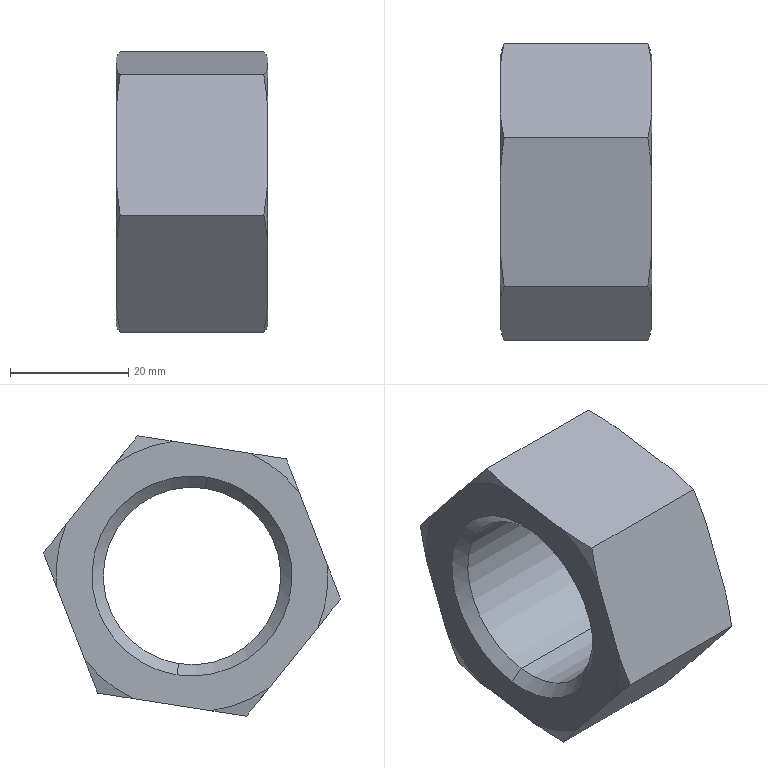Component | SolidWorks | 13Type1HexNut_FinePitch_GradeAAndB[GBT6171-2000][M30_2]-2 | 1 solid | 26 faces | box 25.6 x 50.25 x 47.42 mm | volume 24510 mm3 | cone 16 | plane 8 | cylinder 2 | commonest cylinder face diameters 30 x2 | material Steel
STEP:
#1=CARTESIAN_POINT('',(9.354,-3.462,19.574));
#2=VERTEX_POINT('',#1);
#3=CARTESIAN_POINT('',(9.354,-3.639,20.741));
#4=VERTEX_POINT('',#3);
#5=CARTESIAN_POINT('',(9.354,-3.551,20.157));
#6=DIRECTION('',(-1.,0.,0.));
#7=DIRECTION('',(0.,-0.1496,0.9887));
#8=AXIS2_PLACEMENT_3D('',#5,#6,#7);
#9=CIRCLE('',#8,0.5906);
#10=EDGE_CURVE('',#2,#4,#9,.T.);
#11=ORIENTED_EDGE('',*,*,#10,.F.);
#12=CARTESIAN_POINT('',(9.279,-3.451,19.499));
#13=VERTEX_POINT('',#12);
#14=CARTESIAN_POINT('',(9.354,-3.462,19.574));
#15=DIRECTION('',(-0.7071,0.1058,-0.6991));
#16=VECTOR('',#15,39.37);
#17=LINE('',#14,#16);
#18=EDGE_CURVE('',#2,#13,#17,.T.);
#19=ORIENTED_EDGE('',*,*,#18,.T.);
#20=CARTESIAN_POINT('',(9.279,-3.65,20.816));
#21=VERTEX_POINT('',#20);
#22=CARTESIAN_POINT('',(9.279,-3.551,20.157));
#23=DIRECTION('',(1.,0.,0.));
#24=DIRECTION('',(0.,-0.1496,0.9887));
#25=AXIS2_PLACEMENT_3D('',#22,#23,#24);
#26=CIRCLE('',#25,0.6659);
#27=EDGE_CURVE('',#21,#13,#26,.T.);
#28=ORIENTED_EDGE('',*,*,#27,.F.);
#29=CARTESIAN_POINT('',(9.354,-3.639,20.741));
#30=DIRECTION('',(-0.7071,-0.1058,0.6991));
#31=VECTOR('',#30,39.37);
#32=LINE('',#29,#31);
#33=EDGE_CURVE('',#4,#21,#32,.T.);
#34=ORIENTED_EDGE('',*,*,#33,.F.);
#35=EDGE_LOOP('',(#11,#19,#28,#34));
#36=FACE_OUTER_BOUND('',#35,.T.);
#37=CARTESIAN_POINT('',(9.354,-3.551,20.157));
#38=DIRECTION('',(-1.,0.,0.));
#39=DIRECTION('',(0.,-0.1496,0.9887));
#40=AXIS2_PLACEMENT_3D('',#37,#38,#39);
#41=CONICAL_SURFACE('',#40,0.5906,0.7854);
#42=ADVANCED_FACE('',(#36),#41,.F.);
#43=CARTESIAN_POINT('',(10.211,-3.639,20.741));
#44=VERTEX_POINT('',#43);
#45=CARTESIAN_POINT('',(10.211,-3.462,19.574));
#46=VERTEX_POINT('',#45);
#47=CARTESIAN_POINT('',(10.211,-3.551,20.157));
#48=DIRECTION('',(1.,0.,0.));
#49=DIRECTION('',(0.,-0.1496,0.9887));
#50=AXIS2_PLACEMENT_3D('',#47,#48,#49);
#51=CIRCLE('',#50,0.5906);
#52=EDGE_CURVE('',#44,#46,#51,.T.);
#53=ORIENTED_EDGE('',*,*,#52,.F.);
#54=CARTESIAN_POINT('',(10.287,-3.65,20.816));
#55=VERTEX_POINT('',#54);
#56=CARTESIAN_POINT('',(10.287,-3.65,20.816));
#57=DIRECTION('',(0.7071,-0.1058,0.6991));
#58=VECTOR('',#57,39.37);
#59=LINE('',#56,#58);
#60=EDGE_CURVE('',#44,#55,#59,.T.);
#61=ORIENTED_EDGE('',*,*,#60,.T.);
#62=CARTESIAN_POINT('',(10.287,-3.451,19.499));
#63=VERTEX_POINT('',#62);
#64=CARTESIAN_POINT('',(10.287,-3.551,20.157));
#65=DIRECTION('',(-1.,0.,0.));
#66=DIRECTION('',(0.,-0.1496,0.9887));
#67=AXIS2_PLACEMENT_3D('',#64,#65,#66);
#68=CIRCLE('',#67,0.6659);
#69=EDGE_CURVE('',#63,#55,#68,.T.);
#70=ORIENTED_EDGE('',*,*,#69,.F.);
#71=CARTESIAN_POINT('',(10.287,-3.451,19.499));
#72=DIRECTION('',(0.7071,0.1058,-0.6991));
#73=VECTOR('',#72,39.37);
#74=LINE('',#71,#73);
#75=EDGE_CURVE('',#46,#63,#74,.T.);
#76=ORIENTED_EDGE('',*,*,#75,.F.);
#77=EDGE_LOOP('',(#53,#61,#70,#76));
#78=FACE_OUTER_BOUND('',#77,.T.);
#79=CARTESIAN_POINT('',(10.287,-3.551,20.157));
#80=DIRECTION('',(1.,0.,0.));
#81=DIRECTION('',(0.,0.1496,-0.9887));
#82=AXIS2_PLACEMENT_3D('',#79,#80,#81);
#83=CONICAL_SURFACE('',#82,0.6659,0.7854);
#84=ADVANCED_FACE('',(#78),#83,.F.);
#85=ORIENTED_EDGE('',*,*,#10,.T.);
#86=CARTESIAN_POINT('',(9.279,-3.639,20.741));
#87=DIRECTION('',(1.,0.,0.));
#88=VECTOR('',#87,39.37);
#89=LINE('',#86,#88);
#90=EDGE_CURVE('',#4,#44,#89,.T.);
#91=ORIENTED_EDGE('',*,*,#90,.T.);
#92=ORIENTED_EDGE('',*,*,#52,.T.);
#93=CARTESIAN_POINT('',(9.279,-3.462,19.574));
#94=DIRECTION('',(1.,0.,0.));
#95=VECTOR('',#94,39.37);
#96=LINE('',#93,#95);
#97=EDGE_CURVE('',#2,#46,#96,.T.);
#98=ORIENTED_EDGE('',*,*,#97,.F.);
#99=EDGE_LOOP('',(#85,#91,#92,#98));
#100=FACE_OUTER_BOUND('',#99,.T.);
#101=CARTESIAN_POINT('',(9.279,-3.551,20.157));
#102=DIRECTION('',(1.,0.,0.));
#103=DIRECTION('',(0.,0.1496,-0.9887));
#104=AXIS2_PLACEMENT_3D('',#101,#102,#103);
#105=CYLINDRICAL_SURFACE('',#104,0.5906);
#106=ADVANCED_FACE('',(#100),#105,.F.);
#107=CARTESIAN_POINT('',(9.305,-3.189,21.091));
#108=VERTEX_POINT('',#107);
#109=CARTESIAN_POINT('',(9.279,-3.04,20.905));
#110=VERTEX_POINT('',#109);
#111=CARTESIAN_POINT('',(9.305,-3.189,21.091));
#112=CARTESIAN_POINT('',(9.294,-3.14,21.029));
#113=CARTESIAN_POINT('',(9.285,-3.09,20.967));
#114=CARTESIAN_POINT('',(9.279,-3.04,20.905));
#115=B_SPLINE_CURVE_WITH_KNOTS('',3,(#111,#112,#113,#114),.UNSPECIFIED.,.F.,.F.,(4,4),(0.02506,0.03116),.UNSPECIFIED.);
#116=EDGE_CURVE('',#108,#110,#115,.T.);
#117=ORIENTED_EDGE('',*,*,#116,.F.);
#118=CARTESIAN_POINT('',(10.261,-3.189,21.091));
#119=VERTEX_POINT('',#118);
#120=CARTESIAN_POINT('',(9.279,-3.189,21.091));
#121=DIRECTION('',(1.,0.,0.));
#122=VECTOR('',#121,39.37);
#123=LINE('',#120,#122);
#124=EDGE_CURVE('',#108,#119,#123,.T.);
#125=ORIENTED_EDGE('',*,*,#124,.T.);
#126=CARTESIAN_POINT('',(10.287,-3.04,20.905));
#127=VERTEX_POINT('',#126);
#128=CARTESIAN_POINT('',(10.287,-3.04,20.905));
#129=CARTESIAN_POINT('',(10.281,-3.09,20.967));
#130=CARTESIAN_POINT('',(10.272,-3.14,21.029));
#131=CARTESIAN_POINT('',(10.261,-3.189,21.091));
#132=B_SPLINE_CURVE_WITH_KNOTS('',3,(#128,#129,#130,#131),.UNSPECIFIED.,.F.,.F.,(4,4),(0.04436,0.05035),.UNSPECIFIED.);
#133=EDGE_CURVE('',#127,#119,#132,.T.);
#134=ORIENTED_EDGE('',*,*,#133,.F.);
#135=CARTESIAN_POINT('',(10.287,-2.711,20.497));
#136=VERTEX_POINT('',#135);
#137=CARTESIAN_POINT('',(10.287,-3.189,21.091));
#138=DIRECTION('',(0.,0.627,-0.779));
#139=VECTOR('',#138,39.37);
#140=LINE('',#137,#139);
#141=EDGE_CURVE('',#127,#136,#140,.T.);
#142=ORIENTED_EDGE('',*,*,#141,.T.);
#143=CARTESIAN_POINT('',(10.261,-2.562,20.311));
#144=VERTEX_POINT('',#143);
#145=CARTESIAN_POINT('',(10.261,-2.562,20.311));
#146=CARTESIAN_POINT('',(10.272,-2.611,20.373));
#147=CARTESIAN_POINT('',(10.281,-2.661,20.435));
#148=CARTESIAN_POINT('',(10.287,-2.711,20.497));
#149=B_SPLINE_CURVE_WITH_KNOTS('',3,(#145,#146,#147,#148),.UNSPECIFIED.,.F.,.F.,(4,4),(0.02506,0.03116),.UNSPECIFIED.);
#150=EDGE_CURVE('',#144,#136,#149,.T.);
#151=ORIENTED_EDGE('',*,*,#150,.F.);
#152=CARTESIAN_POINT('',(9.305,-2.562,20.311));
#153=VERTEX_POINT('',#152);
#154=CARTESIAN_POINT('',(9.279,-2.562,20.311));
#155=DIRECTION('',(1.,0.,0.));
#156=VECTOR('',#155,39.37);
#157=LINE('',#154,#156);
#158=EDGE_CURVE('',#153,#144,#157,.T.);
#159=ORIENTED_EDGE('',*,*,#158,.F.);
#160=CARTESIAN_POINT('',(9.279,-2.711,20.497));
#161=VERTEX_POINT('',#160);
#162=CARTESIAN_POINT('',(9.279,-2.711,20.497));
#163=CARTESIAN_POINT('',(9.285,-2.661,20.435));
#164=CARTESIAN_POINT('',(9.294,-2.611,20.373));
#165=CARTESIAN_POINT('',(9.305,-2.562,20.311));
#166=B_SPLINE_CURVE_WITH_KNOTS('',3,(#162,#163,#164,#165),.UNSPECIFIED.,.F.,.F.,(4,4),(0.04436,0.05035),.UNSPECIFIED.);
#167=EDGE_CURVE('',#161,#153,#166,.T.);
#168=ORIENTED_EDGE('',*,*,#167,.F.);
#169=CARTESIAN_POINT('',(9.279,-3.189,21.091));
#170=DIRECTION('',(0.,0.627,-0.779));
#171=VECTOR('',#170,39.37);
#172=LINE('',#169,#171);
#173=EDGE_CURVE('',#110,#161,#172,.T.);
#174=ORIENTED_EDGE('',*,*,#173,.F.);
#175=EDGE_LOOP('',(#117,#125,#134,#142,#151,#159,#168,#174));
#176=FACE_OUTER_BOUND('',#175,.T.);
#177=CARTESIAN_POINT('',(9.279,-3.189,21.091));
#178=DIRECTION('',(0.,-0.779,-0.627));
#179=DIRECTION('',(0.,-0.627,0.779));
#180=AXIS2_PLACEMENT_3D('',#177,#178,#179);
#181=PLANE('',#180);
#182=ADVANCED_FACE('',(#176),#181,.F.);
#183=CARTESIAN_POINT('',(9.279,-2.648,20.088));
#184=VERTEX_POINT('',#183);
#185=CARTESIAN_POINT('',(9.305,-2.562,20.311));
#186=CARTESIAN_POINT('',(9.294,-2.59,20.237));
#187=CARTESIAN_POINT('',(9.285,-2.619,20.163));
#188=CARTESIAN_POINT('',(9.279,-2.648,20.088));
#189=B_SPLINE_CURVE_WITH_KNOTS('',3,(#185,#186,#187,#188),.UNSPECIFIED.,.F.,.F.,(4,4),(0.02495,0.03105),.UNSPECIFIED.);
#190=EDGE_CURVE('',#153,#184,#189,.T.);
#191=ORIENTED_EDGE('',*,*,#190,.F.);
#192=ORIENTED_EDGE('',*,*,#158,.T.);
#193=CARTESIAN_POINT('',(10.287,-2.648,20.088));
#194=VERTEX_POINT('',#193);
#195=CARTESIAN_POINT('',(10.287,-2.648,20.088));
#196=CARTESIAN_POINT('',(10.281,-2.619,20.163));
#197=CARTESIAN_POINT('',(10.272,-2.59,20.237));
#198=CARTESIAN_POINT('',(10.261,-2.562,20.311));
#199=B_SPLINE_CURVE_WITH_KNOTS('',3,(#195,#196,#197,#198),.UNSPECIFIED.,.F.,.F.,(4,4),(0.04424,0.05023),.UNSPECIFIED.);
#200=EDGE_CURVE('',#194,#144,#199,.T.);
#201=ORIENTED_EDGE('',*,*,#200,.F.);
#202=CARTESIAN_POINT('',(10.287,-2.837,19.6));
#203=VERTEX_POINT('',#202);
#204=CARTESIAN_POINT('',(10.287,-2.562,20.311));
#205=DIRECTION('',(0.,-0.3611,-0.9325));
#206=VECTOR('',#205,39.37);
#207=LINE('',#204,#206);
#208=EDGE_CURVE('',#194,#203,#207,.T.);
#209=ORIENTED_EDGE('',*,*,#208,.T.);
#210=CARTESIAN_POINT('',(10.261,-2.923,19.378));
#211=VERTEX_POINT('',#210);
#212=CARTESIAN_POINT('',(10.261,-2.923,19.378));
#213=CARTESIAN_POINT('',(10.272,-2.895,19.452));
#214=CARTESIAN_POINT('',(10.281,-2.866,19.526));
#215=CARTESIAN_POINT('',(10.287,-2.837,19.6));
#216=B_SPLINE_CURVE_WITH_KNOTS('',3,(#212,#213,#214,#215),.UNSPECIFIED.,.F.,.F.,(4,4),(0.02495,0.03105),.UNSPECIFIED.);
#217=EDGE_CURVE('',#211,#203,#216,.T.);
#218=ORIENTED_EDGE('',*,*,#217,.F.);
#219=CARTESIAN_POINT('',(9.305,-2.923,19.378));
#220=VERTEX_POINT('',#219);
#221=CARTESIAN_POINT('',(9.279,-2.923,19.378));
#222=DIRECTION('',(1.,0.,0.));
#223=VECTOR('',#222,39.37);
#224=LINE('',#221,#223);
#225=EDGE_CURVE('',#220,#211,#224,.T.);
#226=ORIENTED_EDGE('',*,*,#225,.F.);
#227=CARTESIAN_POINT('',(9.279,-2.837,19.6));
#228=VERTEX_POINT('',#227);
#229=CARTESIAN_POINT('',(9.279,-2.837,19.6));
#230=CARTESIAN_POINT('',(9.285,-2.866,19.526));
#231=CARTESIAN_POINT('',(9.294,-2.895,19.452));
#232=CARTESIAN_POINT('',(9.305,-2.923,19.378));
#233=B_SPLINE_CURVE_WITH_KNOTS('',3,(#229,#230,#231,#232),.UNSPECIFIED.,.F.,.F.,(4,4),(0.04424,0.05023),.UNSPECIFIED.);
#234=EDGE_CURVE('',#228,#220,#233,.T.);
#235=ORIENTED_EDGE('',*,*,#234,.F.);
#236=CARTESIAN_POINT('',(9.279,-2.562,20.311));
#237=DIRECTION('',(0.,-0.3611,-0.9325));
#238=VECTOR('',#237,39.37);
#239=LINE('',#236,#238);
#240=EDGE_CURVE('',#184,#228,#239,.T.);
#241=ORIENTED_EDGE('',*,*,#240,.F.);
#242=EDGE_LOOP('',(#191,#192,#201,#209,#218,#226,#235,#241));
#243=FACE_OUTER_BOUND('',#242,.T.);
#244=CARTESIAN_POINT('',(9.279,-2.562,20.311));
#245=DIRECTION('',(0.,-0.9325,0.3611));
#246=DIRECTION('',(0.,0.3611,0.9325));
#247=AXIS2_PLACEMENT_3D('',#244,#245,#246);
#248=PLANE('',#247);
#249=ADVANCED_FACE('',(#243),#248,.F.);
#250=CARTESIAN_POINT('',(9.279,-3.159,19.341));
#251=VERTEX_POINT('',#250);
#252=CARTESIAN_POINT('',(9.305,-2.923,19.378));
#253=CARTESIAN_POINT('',(9.294,-3.002,19.366));
#254=CARTESIAN_POINT('',(9.285,-3.08,19.353));
#255=CARTESIAN_POINT('',(9.279,-3.159,19.341));
#256=B_SPLINE_CURVE_WITH_KNOTS('',3,(#252,#253,#254,#255),.UNSPECIFIED.,.F.,.F.,(4,4),(0.02163,0.02773),.UNSPECIFIED.);
#257=EDGE_CURVE('',#220,#251,#256,.T.);
#258=ORIENTED_EDGE('',*,*,#257,.F.);
#259=ORIENTED_EDGE('',*,*,#225,.T.);
#260=CARTESIAN_POINT('',(10.287,-3.159,19.341));
#261=VERTEX_POINT('',#260);
#262=CARTESIAN_POINT('',(10.287,-3.159,19.341));
#263=CARTESIAN_POINT('',(10.284,-3.12,19.347));
#264=CARTESIAN_POINT('',(10.28,-3.08,19.353));
#265=CARTESIAN_POINT('',(10.271,-3.002,19.366));
#266=CARTESIAN_POINT('',(10.267,-2.962,19.372));
#267=CARTESIAN_POINT('',(10.261,-2.923,19.378));
#268=B_SPLINE_CURVE_WITH_KNOTS('',3,(#262,#263,#264,#265,#266,#267),.UNSPECIFIED.,.F.,.F.,(4,2,4),(0.04094,0.04393,0.04693),.UNSPECIFIED.);
#269=EDGE_CURVE('',#261,#211,#268,.T.);
#270=ORIENTED_EDGE('',*,*,#269,.F.);
#271=CARTESIAN_POINT('',(10.287,-3.676,19.261));
#272=VERTEX_POINT('',#271);
#273=CARTESIAN_POINT('',(10.287,-2.923,19.378));
#274=DIRECTION('',(0.,-0.9881,-0.1535));
#275=VECTOR('',#274,39.37);
#276=LINE('',#273,#275);
#277=EDGE_CURVE('',#261,#272,#276,.T.);
#278=ORIENTED_EDGE('',*,*,#277,.T.);
#279=CARTESIAN_POINT('',(10.261,-3.912,19.224));
#280=VERTEX_POINT('',#279);
#281=CARTESIAN_POINT('',(10.261,-3.912,19.224));
#282=CARTESIAN_POINT('',(10.272,-3.834,19.236));
#283=CARTESIAN_POINT('',(10.281,-3.755,19.248));
#284=CARTESIAN_POINT('',(10.287,-3.676,19.261));
#285=B_SPLINE_CURVE_WITH_KNOTS('',3,(#281,#282,#283,#284),.UNSPECIFIED.,.F.,.F.,(4,4),(0.02163,0.02773),.UNSPECIFIED.);
#286=EDGE_CURVE('',#280,#272,#285,.T.);
#287=ORIENTED_EDGE('',*,*,#286,.F.);
#288=CARTESIAN_POINT('',(9.305,-3.912,19.224));
#289=VERTEX_POINT('',#288);
#290=CARTESIAN_POINT('',(9.279,-3.912,19.224));
#291=DIRECTION('',(1.,0.,0.));
#292=VECTOR('',#291,39.37);
#293=LINE('',#290,#292);
#294=EDGE_CURVE('',#289,#280,#293,.T.);
#295=ORIENTED_EDGE('',*,*,#294,.F.);
#296=CARTESIAN_POINT('',(9.279,-3.676,19.261));
#297=VERTEX_POINT('',#296);
#298=CARTESIAN_POINT('',(9.279,-3.676,19.261));
#299=CARTESIAN_POINT('',(9.282,-3.716,19.255));
#300=CARTESIAN_POINT('',(9.286,-3.755,19.248));
#301=CARTESIAN_POINT('',(9.294,-3.834,19.236));
#302=CARTESIAN_POINT('',(9.299,-3.873,19.23));
#303=CARTESIAN_POINT('',(9.305,-3.912,19.224));
#304=B_SPLINE_CURVE_WITH_KNOTS('',3,(#298,#299,#300,#301,#302,#303),.UNSPECIFIED.,.F.,.F.,(4,2,4),(0.04094,0.04393,0.04693),.UNSPECIFIED.);
#305=EDGE_CURVE('',#297,#289,#304,.T.);
#306=ORIENTED_EDGE('',*,*,#305,.F.);
#307=CARTESIAN_POINT('',(9.279,-2.923,19.378));
#308=DIRECTION('',(0.,-0.9881,-0.1535));
#309=VECTOR('',#308,39.37);
#310=LINE('',#307,#309);
#311=EDGE_CURVE('',#251,#297,#310,.T.);
#312=ORIENTED_EDGE('',*,*,#311,.F.);
#313=EDGE_LOOP('',(#258,#259,#270,#278,#287,#295,#306,#312));
#314=FACE_OUTER_BOUND('',#313,.T.);
#315=CARTESIAN_POINT('',(9.279,-2.923,19.378));
#316=DIRECTION('',(0.,-0.1535,0.9881));
#317=DIRECTION('',(0.,0.9881,0.1535));
#318=AXIS2_PLACEMENT_3D('',#315,#316,#317);
#319=PLANE('',#318);
#320=ADVANCED_FACE('',(#314),#319,.F.);
#321=CARTESIAN_POINT('',(9.279,-4.062,19.41));
#322=VERTEX_POINT('',#321);
#323=CARTESIAN_POINT('',(9.305,-3.912,19.224));
#324=CARTESIAN_POINT('',(9.294,-3.962,19.286));
#325=CARTESIAN_POINT('',(9.285,-4.012,19.348));
#326=CARTESIAN_POINT('',(9.279,-4.062,19.41));
#327=B_SPLINE_CURVE_WITH_KNOTS('',3,(#323,#324,#325,#326),.UNSPECIFIED.,.F.,.F.,(4,4),(0.02506,0.03116),.UNSPECIFIED.);
#328=EDGE_CURVE('',#289,#322,#327,.T.);
#329=ORIENTED_EDGE('',*,*,#328,.F.);
#330=ORIENTED_EDGE('',*,*,#294,.T.);
#331=CARTESIAN_POINT('',(10.287,-4.062,19.41));
#332=VERTEX_POINT('',#331);
#333=CARTESIAN_POINT('',(10.287,-4.062,19.41));
#334=CARTESIAN_POINT('',(10.281,-4.012,19.348));
#335=CARTESIAN_POINT('',(10.272,-3.962,19.286));
#336=CARTESIAN_POINT('',(10.261,-3.912,19.224));
#337=B_SPLINE_CURVE_WITH_KNOTS('',3,(#333,#334,#335,#336),.UNSPECIFIED.,.F.,.F.,(4,4),(0.04436,0.05035),.UNSPECIFIED.);
#338=EDGE_CURVE('',#332,#280,#337,.T.);
#339=ORIENTED_EDGE('',*,*,#338,.F.);
#340=CARTESIAN_POINT('',(10.287,-4.39,19.818));
#341=VERTEX_POINT('',#340);
#342=CARTESIAN_POINT('',(10.287,-3.912,19.224));
#343=DIRECTION('',(0.,-0.627,0.779));
#344=VECTOR('',#343,39.37);
#345=LINE('',#342,#344);
#346=EDGE_CURVE('',#332,#341,#345,.T.);
#347=ORIENTED_EDGE('',*,*,#346,.T.);
#348=CARTESIAN_POINT('',(10.261,-4.54,20.004));
#349=VERTEX_POINT('',#348);
#350=CARTESIAN_POINT('',(10.261,-4.54,20.004));
#351=CARTESIAN_POINT('',(10.272,-4.49,19.942));
#352=CARTESIAN_POINT('',(10.281,-4.44,19.88));
#353=CARTESIAN_POINT('',(10.287,-4.39,19.818));
#354=B_SPLINE_CURVE_WITH_KNOTS('',3,(#350,#351,#352,#353),.UNSPECIFIED.,.F.,.F.,(4,4),(0.02506,0.03116),.UNSPECIFIED.);
#355=EDGE_CURVE('',#349,#341,#354,.T.);
#356=ORIENTED_EDGE('',*,*,#355,.F.);
#357=CARTESIAN_POINT('',(9.305,-4.54,20.004));
#358=VERTEX_POINT('',#357);
#359=CARTESIAN_POINT('',(9.279,-4.54,20.004));
#360=DIRECTION('',(1.,0.,0.));
#361=VECTOR('',#360,39.37);
#362=LINE('',#359,#361);
#363=EDGE_CURVE('',#358,#349,#362,.T.);
#364=ORIENTED_EDGE('',*,*,#363,.F.);
#365=CARTESIAN_POINT('',(9.279,-4.39,19.818));
#366=VERTEX_POINT('',#365);
#367=CARTESIAN_POINT('',(9.279,-4.39,19.818));
#368=CARTESIAN_POINT('',(9.285,-4.44,19.88));
#369=CARTESIAN_POINT('',(9.294,-4.49,19.942));
#370=CARTESIAN_POINT('',(9.305,-4.54,20.004));
#371=B_SPLINE_CURVE_WITH_KNOTS('',3,(#367,#368,#369,#370),.UNSPECIFIED.,.F.,.F.,(4,4),(0.04436,0.05035),.UNSPECIFIED.);
#372=EDGE_CURVE('',#366,#358,#371,.T.);
#373=ORIENTED_EDGE('',*,*,#372,.F.);
#374=CARTESIAN_POINT('',(9.279,-3.912,19.224));
#375=DIRECTION('',(0.,-0.627,0.779));
#376=VECTOR('',#375,39.37);
#377=LINE('',#374,#376);
#378=EDGE_CURVE('',#322,#366,#377,.T.);
#379=ORIENTED_EDGE('',*,*,#378,.F.);
#380=EDGE_LOOP('',(#329,#330,#339,#347,#356,#364,#373,#379));
#381=FACE_OUTER_BOUND('',#380,.T.);
#382=CARTESIAN_POINT('',(9.279,-3.912,19.224));
#383=DIRECTION('',(0.,0.779,0.627));
#384=DIRECTION('',(0.,0.627,-0.779));
#385=AXIS2_PLACEMENT_3D('',#382,#383,#384);
#386=PLANE('',#385);
#387=ADVANCED_FACE('',(#381),#386,.F.);
#388=CARTESIAN_POINT('',(9.279,-4.454,20.227));
#389=VERTEX_POINT('',#388);
#390=CARTESIAN_POINT('',(9.305,-4.54,20.004));
#391=CARTESIAN_POINT('',(9.294,-4.511,20.078));
#392=CARTESIAN_POINT('',(9.285,-4.483,20.152));
#393=CARTESIAN_POINT('',(9.279,-4.454,20.227));
#394=B_SPLINE_CURVE_WITH_KNOTS('',3,(#390,#391,#392,#393),.UNSPECIFIED.,.F.,.F.,(4,4),(0.02495,0.03105),.UNSPECIFIED.);
#395=EDGE_CURVE('',#358,#389,#394,.T.);
#396=ORIENTED_EDGE('',*,*,#395,.F.);
#397=ORIENTED_EDGE('',*,*,#363,.T.);
#398=CARTESIAN_POINT('',(10.287,-4.454,20.227));
#399=VERTEX_POINT('',#398);
#400=CARTESIAN_POINT('',(10.287,-4.454,20.227));
#401=CARTESIAN_POINT('',(10.281,-4.483,20.152));
#402=CARTESIAN_POINT('',(10.272,-4.511,20.078));
#403=CARTESIAN_POINT('',(10.261,-4.54,20.004));
#404=B_SPLINE_CURVE_WITH_KNOTS('',3,(#400,#401,#402,#403),.UNSPECIFIED.,.F.,.F.,(4,4),(0.04424,0.05023),.UNSPECIFIED.);
#405=EDGE_CURVE('',#399,#349,#404,.T.);
#406=ORIENTED_EDGE('',*,*,#405,.F.);
#407=CARTESIAN_POINT('',(10.287,-4.265,20.715));
#408=VERTEX_POINT('',#407);
#409=CARTESIAN_POINT('',(10.287,-4.54,20.004));
#410=DIRECTION('',(0.,0.3611,0.9325));
#411=VECTOR('',#410,39.37);
#412=LINE('',#409,#411);
#413=EDGE_CURVE('',#399,#408,#412,.T.);
#414=ORIENTED_EDGE('',*,*,#413,.T.);
#415=CARTESIAN_POINT('',(10.261,-4.178,20.937));
#416=VERTEX_POINT('',#415);
#417=CARTESIAN_POINT('',(10.261,-4.178,20.937));
#418=CARTESIAN_POINT('',(10.272,-4.207,20.863));
#419=CARTESIAN_POINT('',(10.281,-4.236,20.789));
#420=CARTESIAN_POINT('',(10.287,-4.265,20.715));
#421=B_SPLINE_CURVE_WITH_KNOTS('',3,(#417,#418,#419,#420),.UNSPECIFIED.,.F.,.F.,(4,4),(0.02495,0.03105),.UNSPECIFIED.);
#422=EDGE_CURVE('',#416,#408,#421,.T.);
#423=ORIENTED_EDGE('',*,*,#422,.F.);
#424=CARTESIAN_POINT('',(9.305,-4.178,20.937));
#425=VERTEX_POINT('',#424);
#426=CARTESIAN_POINT('',(9.279,-4.178,20.937));
#427=DIRECTION('',(1.,0.,0.));
#428=VECTOR('',#427,39.37);
#429=LINE('',#426,#428);
#430=EDGE_CURVE('',#425,#416,#429,.T.);
#431=ORIENTED_EDGE('',*,*,#430,.F.);
#432=CARTESIAN_POINT('',(9.279,-4.265,20.715));
#433=VERTEX_POINT('',#432);
#434=CARTESIAN_POINT('',(9.279,-4.265,20.715));
#435=CARTESIAN_POINT('',(9.285,-4.236,20.789));
#436=CARTESIAN_POINT('',(9.294,-4.207,20.863));
#437=CARTESIAN_POINT('',(9.305,-4.178,20.937));
#438=B_SPLINE_CURVE_WITH_KNOTS('',3,(#434,#435,#436,#437),.UNSPECIFIED.,.F.,.F.,(4,4),(0.04424,0.05023),.UNSPECIFIED.);
#439=EDGE_CURVE('',#433,#425,#438,.T.);
#440=ORIENTED_EDGE('',*,*,#439,.F.);
#441=CARTESIAN_POINT('',(9.279,-4.54,20.004));
#442=DIRECTION('',(0.,0.3611,0.9325));
#443=VECTOR('',#442,39.37);
#444=LINE('',#441,#443);
#445=EDGE_CURVE('',#389,#433,#444,.T.);
#446=ORIENTED_EDGE('',*,*,#445,.F.);
#447=EDGE_LOOP('',(#396,#397,#406,#414,#423,#431,#440,#446));
#448=FACE_OUTER_BOUND('',#447,.T.);
#449=CARTESIAN_POINT('',(9.279,-4.54,20.004));
#450=DIRECTION('',(0.,0.9325,-0.3611));
#451=DIRECTION('',(0.,-0.3611,-0.9325));
#452=AXIS2_PLACEMENT_3D('',#449,#450,#451);
#453=PLANE('',#452);
#454=ADVANCED_FACE('',(#448),#453,.F.);
#455=CARTESIAN_POINT('',(9.279,-3.942,20.974));
#456=VERTEX_POINT('',#455);
#457=CARTESIAN_POINT('',(9.305,-4.178,20.937));
#458=CARTESIAN_POINT('',(9.294,-4.1,20.949));
#459=CARTESIAN_POINT('',(9.285,-4.021,20.962));
#460=CARTESIAN_POINT('',(9.279,-3.942,20.974));
#461=B_SPLINE_CURVE_WITH_KNOTS('',3,(#457,#458,#459,#460),.UNSPECIFIED.,.F.,.F.,(4,4),(0.02163,0.02773),.UNSPECIFIED.);
#462=EDGE_CURVE('',#425,#456,#461,.T.);
#463=ORIENTED_EDGE('',*,*,#462,.F.);
#464=ORIENTED_EDGE('',*,*,#430,.T.);
#465=CARTESIAN_POINT('',(10.287,-3.942,20.974));
#466=VERTEX_POINT('',#465);
#467=CARTESIAN_POINT('',(10.287,-3.942,20.974));
#468=CARTESIAN_POINT('',(10.284,-3.982,20.968));
#469=CARTESIAN_POINT('',(10.28,-4.021,20.962));
#470=CARTESIAN_POINT('',(10.271,-4.1,20.949));
#471=CARTESIAN_POINT('',(10.267,-4.139,20.943));
#472=CARTESIAN_POINT('',(10.261,-4.178,20.937));
#473=B_SPLINE_CURVE_WITH_KNOTS('',3,(#467,#468,#469,#470,#471,#472),.UNSPECIFIED.,.F.,.F.,(4,2,4),(0.04094,0.04393,0.04693),.UNSPECIFIED.);
#474=EDGE_CURVE('',#466,#416,#473,.T.);
#475=ORIENTED_EDGE('',*,*,#474,.F.);
#476=CARTESIAN_POINT('',(10.287,-3.425,21.054));
#477=VERTEX_POINT('',#476);
#478=CARTESIAN_POINT('',(10.287,-4.178,20.937));
#479=DIRECTION('',(0.,0.9881,0.1535));
#480=VECTOR('',#479,39.37);
#481=LINE('',#478,#480);
#482=EDGE_CURVE('',#466,#477,#481,.T.);
#483=ORIENTED_EDGE('',*,*,#482,.T.);
#484=CARTESIAN_POINT('',(10.261,-3.189,21.091));
#485=CARTESIAN_POINT('',(10.272,-3.268,21.079));
#486=CARTESIAN_POINT('',(10.281,-3.346,21.067));
#487=CARTESIAN_POINT('',(10.287,-3.425,21.054));
#488=B_SPLINE_CURVE_WITH_KNOTS('',3,(#484,#485,#486,#487),.UNSPECIFIED.,.F.,.F.,(4,4),(0.02163,0.02773),.UNSPECIFIED.);
#489=EDGE_CURVE('',#119,#477,#488,.T.);
#490=ORIENTED_EDGE('',*,*,#489,.F.);
#491=ORIENTED_EDGE('',*,*,#124,.F.);
#492=CARTESIAN_POINT('',(9.279,-3.425,21.054));
#493=VERTEX_POINT('',#492);
#494=CARTESIAN_POINT('',(9.279,-3.425,21.054));
#495=CARTESIAN_POINT('',(9.282,-3.386,21.06));
#496=CARTESIAN_POINT('',(9.286,-3.346,21.067));
#497=CARTESIAN_POINT('',(9.294,-3.268,21.079));
#498=CARTESIAN_POINT('',(9.299,-3.229,21.085));
#499=CARTESIAN_POINT('',(9.305,-3.189,21.091));
#500=B_SPLINE_CURVE_WITH_KNOTS('',3,(#494,#495,#496,#497,#498,#499),.UNSPECIFIED.,.F.,.F.,(4,2,4),(0.04094,0.04393,0.04693),.UNSPECIFIED.);
#501=EDGE_CURVE('',#493,#108,#500,.T.);
#502=ORIENTED_EDGE('',*,*,#501,.F.);
#503=CARTESIAN_POINT('',(9.279,-4.178,20.937));
#504=DIRECTION('',(0.,0.9881,0.1535));
#505=VECTOR('',#504,39.37);
#506=LINE('',#503,#505);
#507=EDGE_CURVE('',#456,#493,#506,.T.);
#508=ORIENTED_EDGE('',*,*,#507,.F.);
#509=EDGE_LOOP('',(#463,#464,#475,#483,#490,#491,#502,#508));
#510=FACE_OUTER_BOUND('',#509,.T.);
#511=CARTESIAN_POINT('',(9.279,-4.178,20.937));
#512=DIRECTION('',(0.,0.1535,-0.9881));
#513=DIRECTION('',(0.,-0.9881,-0.1535));
#514=AXIS2_PLACEMENT_3D('',#511,#512,#513);
#515=PLANE('',#514);
#516=ADVANCED_FACE('',(#510),#515,.F.);
#517=ORIENTED_EDGE('',*,*,#27,.T.);
#518=CARTESIAN_POINT('',(9.279,-3.551,20.157));
#519=DIRECTION('',(1.,0.,0.));
#520=DIRECTION('',(0.,-0.1496,0.9887));
#521=AXIS2_PLACEMENT_3D('',#518,#519,#520);
#522=CIRCLE('',#521,0.6659);
#523=EDGE_CURVE('',#13,#21,#522,.T.);
#524=ORIENTED_EDGE('',*,*,#523,.T.);
#525=EDGE_LOOP('',(#517,#524));
#526=FACE_BOUND('',#525,.T.);
#527=ORIENTED_EDGE('',*,*,#507,.T.);
#528=CARTESIAN_POINT('',(9.279,-3.551,20.157));
#529=DIRECTION('',(-1.,0.,0.));
#530=DIRECTION('',(0.,-0.1496,0.9887));
#531=AXIS2_PLACEMENT_3D('',#528,#529,#530);
#532=CIRCLE('',#531,0.9055);
#533=EDGE_CURVE('',#493,#110,#532,.T.);
#534=ORIENTED_EDGE('',*,*,#533,.T.);
#535=ORIENTED_EDGE('',*,*,#173,.T.);
#536=CARTESIAN_POINT('',(9.279,-3.551,20.157));
#537=DIRECTION('',(-1.,0.,0.));
#538=DIRECTION('',(0.,-0.1496,0.9887));
#539=AXIS2_PLACEMENT_3D('',#536,#537,#538);
#540=CIRCLE('',#539,0.9055);
#541=EDGE_CURVE('',#161,#184,#540,.T.);
#542=ORIENTED_EDGE('',*,*,#541,.T.);
#543=ORIENTED_EDGE('',*,*,#240,.T.);
#544=CARTESIAN_POINT('',(9.279,-3.551,20.157));
#545=DIRECTION('',(-1.,0.,0.));
#546=DIRECTION('',(0.,-0.1496,0.9887));
#547=AXIS2_PLACEMENT_3D('',#544,#545,#546);
#548=CIRCLE('',#547,0.9055);
#549=EDGE_CURVE('',#228,#251,#548,.T.);
#550=ORIENTED_EDGE('',*,*,#549,.T.);
#551=ORIENTED_EDGE('',*,*,#311,.T.);
#552=CARTESIAN_POINT('',(9.279,-3.551,20.157));
#553=DIRECTION('',(-1.,0.,0.));
#554=DIRECTION('',(0.,-0.1496,0.9887));
#555=AXIS2_PLACEMENT_3D('',#552,#553,#554);
#556=CIRCLE('',#555,0.9055);
#557=EDGE_CURVE('',#297,#322,#556,.T.);
#558=ORIENTED_EDGE('',*,*,#557,.T.);
#559=ORIENTED_EDGE('',*,*,#378,.T.);
#560=CARTESIAN_POINT('',(9.279,-3.551,20.157));
#561=DIRECTION('',(-1.,0.,0.));
#562=DIRECTION('',(0.,-0.1496,0.9887));
#563=AXIS2_PLACEMENT_3D('',#560,#561,#562);
#564=CIRCLE('',#563,0.9055);
#565=EDGE_CURVE('',#366,#389,#564,.T.);
#566=ORIENTED_EDGE('',*,*,#565,.T.);
#567=ORIENTED_EDGE('',*,*,#445,.T.);
#568=CARTESIAN_POINT('',(9.279,-3.551,20.157));
#569=DIRECTION('',(-1.,0.,0.));
#570=DIRECTION('',(0.,-0.1496,0.9887));
#571=AXIS2_PLACEMENT_3D('',#568,#569,#570);
#572=CIRCLE('',#571,0.9055);
#573=EDGE_CURVE('',#433,#456,#572,.T.);
#574=ORIENTED_EDGE('',*,*,#573,.T.);
#575=EDGE_LOOP('',(#527,#534,#535,#542,#543,#550,#551,#558,#559,#566,#567,#574));
#576=FACE_OUTER_BOUND('',#575,.T.);
#577=CARTESIAN_POINT('',(9.279,-2.562,20.311));
#578=DIRECTION('',(-1.,0.,0.));
#579=DIRECTION('',(0.,-0.1496,0.9887));
#580=AXIS2_PLACEMENT_3D('',#577,#578,#579);
#581=PLANE('',#580);
#582=ADVANCED_FACE('',(#526,#576),#581,.T.);
#583=ORIENTED_EDGE('',*,*,#69,.T.);
#584=CARTESIAN_POINT('',(10.287,-3.551,20.157));
#585=DIRECTION('',(-1.,0.,0.));
#586=DIRECTION('',(0.,-0.1496,0.9887));
#587=AXIS2_PLACEMENT_3D('',#584,#585,#586);
#588=CIRCLE('',#587,0.6659);
#589=EDGE_CURVE('',#55,#63,#588,.T.);
#590=ORIENTED_EDGE('',*,*,#589,.T.);
#591=EDGE_LOOP('',(#583,#590));
#592=FACE_BOUND('',#591,.T.);
#593=CARTESIAN_POINT('',(10.287,-3.551,20.157));
#594=DIRECTION('',(1.,0.,0.));
#595=DIRECTION('',(0.,0.1496,-0.9887));
#596=AXIS2_PLACEMENT_3D('',#593,#594,#595);
#597=CIRCLE('',#596,0.9055);
#598=EDGE_CURVE('',#127,#477,#597,.T.);
#599=ORIENTED_EDGE('',*,*,#598,.T.);
#600=ORIENTED_EDGE('',*,*,#482,.F.);
#601=CARTESIAN_POINT('',(10.287,-3.551,20.157));
#602=DIRECTION('',(1.,0.,0.));
#603=DIRECTION('',(0.,0.1496,-0.9887));
#604=AXIS2_PLACEMENT_3D('',#601,#602,#603);
#605=CIRCLE('',#604,0.9055);
#606=EDGE_CURVE('',#466,#408,#605,.T.);
#607=ORIENTED_EDGE('',*,*,#606,.T.);
#608=ORIENTED_EDGE('',*,*,#413,.F.);
#609=CARTESIAN_POINT('',(10.287,-3.551,20.157));
#610=DIRECTION('',(1.,0.,0.));
#611=DIRECTION('',(0.,0.1496,-0.9887));
#612=AXIS2_PLACEMENT_3D('',#609,#610,#611);
#613=CIRCLE('',#612,0.9055);
#614=EDGE_CURVE('',#399,#341,#613,.T.);
#615=ORIENTED_EDGE('',*,*,#614,.T.);
#616=ORIENTED_EDGE('',*,*,#346,.F.);
#617=CARTESIAN_POINT('',(10.287,-3.551,20.157));
#618=DIRECTION('',(1.,0.,0.));
#619=DIRECTION('',(0.,0.1496,-0.9887));
#620=AXIS2_PLACEMENT_3D('',#617,#618,#619);
#621=CIRCLE('',#620,0.9055);
#622=EDGE_CURVE('',#332,#272,#621,.T.);
#623=ORIENTED_EDGE('',*,*,#622,.T.);
#624=ORIENTED_EDGE('',*,*,#277,.F.);
#625=CARTESIAN_POINT('',(10.287,-3.551,20.157));
#626=DIRECTION('',(1.,0.,0.));
#627=DIRECTION('',(0.,0.1496,-0.9887));
#628=AXIS2_PLACEMENT_3D('',#625,#626,#627);
#629=CIRCLE('',#628,0.9055);
#630=EDGE_CURVE('',#261,#203,#629,.T.);
#631=ORIENTED_EDGE('',*,*,#630,.T.);
#632=ORIENTED_EDGE('',*,*,#208,.F.);
#633=CARTESIAN_POINT('',(10.287,-3.551,20.157));
#634=DIRECTION('',(1.,0.,0.));
#635=DIRECTION('',(0.,0.1496,-0.9887));
#636=AXIS2_PLACEMENT_3D('',#633,#634,#635);
#637=CIRCLE('',#636,0.9055);
#638=EDGE_CURVE('',#194,#136,#637,.T.);
#639=ORIENTED_EDGE('',*,*,#638,.T.);
#640=ORIENTED_EDGE('',*,*,#141,.F.);
#641=EDGE_LOOP('',(#599,#600,#607,#608,#615,#616,#623,#624,#631,#632,#639,#640));
#642=FACE_OUTER_BOUND('',#641,.T.);
#643=CARTESIAN_POINT('',(10.287,-2.562,20.311));
#644=DIRECTION('',(-1.,0.,0.));
#645=DIRECTION('',(0.,-0.1496,0.9887));
#646=AXIS2_PLACEMENT_3D('',#643,#644,#645);
#647=PLANE('',#646);
#648=ADVANCED_FACE('',(#592,#642),#647,.F.);
#649=ORIENTED_EDGE('',*,*,#90,.F.);
#650=CARTESIAN_POINT('',(9.354,-3.551,20.157));
#651=DIRECTION('',(-1.,0.,0.));
#652=DIRECTION('',(0.,-0.1496,0.9887));
#653=AXIS2_PLACEMENT_3D('',#650,#651,#652);
#654=CIRCLE('',#653,0.5906);
#655=EDGE_CURVE('',#4,#2,#654,.T.);
#656=ORIENTED_EDGE('',*,*,#655,.T.);
#657=ORIENTED_EDGE('',*,*,#97,.T.);
#658=CARTESIAN_POINT('',(10.211,-3.551,20.157));
#659=DIRECTION('',(1.,0.,0.));
#660=DIRECTION('',(0.,-0.1496,0.9887));
#661=AXIS2_PLACEMENT_3D('',#658,#659,#660);
#662=CIRCLE('',#661,0.5906);
#663=EDGE_CURVE('',#46,#44,#662,.T.);
#664=ORIENTED_EDGE('',*,*,#663,.T.);
#665=EDGE_LOOP('',(#649,#656,#657,#664));
#666=FACE_OUTER_BOUND('',#665,.T.);
#667=CARTESIAN_POINT('',(9.279,-3.551,20.157));
#668=DIRECTION('',(1.,0.,0.));
#669=DIRECTION('',(0.,0.1496,-0.9887));
#670=AXIS2_PLACEMENT_3D('',#667,#668,#669);
#671=CYLINDRICAL_SURFACE('',#670,0.5906);
#672=ADVANCED_FACE('',(#666),#671,.F.);
#673=ORIENTED_EDGE('',*,*,#422,.T.);
#674=ORIENTED_EDGE('',*,*,#606,.F.);
#675=ORIENTED_EDGE('',*,*,#474,.T.);
#676=EDGE_LOOP('',(#673,#674,#675));
#677=FACE_OUTER_BOUND('',#676,.T.);
#678=CARTESIAN_POINT('',(10.287,-3.551,20.157));
#679=DIRECTION('',(-1.,0.,0.));
#680=DIRECTION('',(0.,0.1496,-0.9887));
#681=AXIS2_PLACEMENT_3D('',#678,#679,#680);
#682=CONICAL_SURFACE('',#681,0.9055,1.309);
#683=ADVANCED_FACE('',(#677),#682,.T.);
#684=ORIENTED_EDGE('',*,*,#133,.T.);
#685=ORIENTED_EDGE('',*,*,#489,.T.);
#686=ORIENTED_EDGE('',*,*,#598,.F.);
#687=EDGE_LOOP('',(#684,#685,#686));
#688=FACE_OUTER_BOUND('',#687,.T.);
#689=CARTESIAN_POINT('',(10.287,-3.551,20.157));
#690=DIRECTION('',(-1.,0.,0.));
#691=DIRECTION('',(0.,0.1496,-0.9887));
#692=AXIS2_PLACEMENT_3D('',#689,#690,#691);
#693=CONICAL_SURFACE('',#692,0.9055,1.309);
#694=ADVANCED_FACE('',(#688),#693,.T.);
#695=ORIENTED_EDGE('',*,*,#355,.T.);
#696=ORIENTED_EDGE('',*,*,#614,.F.);
#697=ORIENTED_EDGE('',*,*,#405,.T.);
#698=EDGE_LOOP('',(#695,#696,#697));
#699=FACE_OUTER_BOUND('',#698,.T.);
#700=CARTESIAN_POINT('',(10.287,-3.551,20.157));
#701=DIRECTION('',(-1.,0.,0.));
#702=DIRECTION('',(0.,0.1496,-0.9887));
#703=AXIS2_PLACEMENT_3D('',#700,#701,#702);
#704=CONICAL_SURFACE('',#703,0.9055,1.309);
#705=ADVANCED_FACE('',(#699),#704,.T.);
#706=ORIENTED_EDGE('',*,*,#286,.T.);
#707=ORIENTED_EDGE('',*,*,#622,.F.);
#708=ORIENTED_EDGE('',*,*,#338,.T.);
#709=EDGE_LOOP('',(#706,#707,#708));
#710=FACE_OUTER_BOUND('',#709,.T.);
#711=CARTESIAN_POINT('',(10.287,-3.551,20.157));
#712=DIRECTION('',(-1.,0.,0.));
#713=DIRECTION('',(0.,0.1496,-0.9887));
#714=AXIS2_PLACEMENT_3D('',#711,#712,#713);
#715=CONICAL_SURFACE('',#714,0.9055,1.309);
#716=ADVANCED_FACE('',(#710),#715,.T.);
#717=ORIENTED_EDGE('',*,*,#217,.T.);
#718=ORIENTED_EDGE('',*,*,#630,.F.);
#719=ORIENTED_EDGE('',*,*,#269,.T.);
#720=EDGE_LOOP('',(#717,#718,#719));
#721=FACE_OUTER_BOUND('',#720,.T.);
#722=CARTESIAN_POINT('',(10.287,-3.551,20.157));
#723=DIRECTION('',(-1.,0.,0.));
#724=DIRECTION('',(0.,0.1496,-0.9887));
#725=AXIS2_PLACEMENT_3D('',#722,#723,#724);
#726=CONICAL_SURFACE('',#725,0.9055,1.309);
#727=ADVANCED_FACE('',(#721),#726,.T.);
#728=ORIENTED_EDGE('',*,*,#150,.T.);
#729=ORIENTED_EDGE('',*,*,#638,.F.);
#730=ORIENTED_EDGE('',*,*,#200,.T.);
#731=EDGE_LOOP('',(#728,#729,#730));
#732=FACE_OUTER_BOUND('',#731,.T.);
#733=CARTESIAN_POINT('',(10.287,-3.551,20.157));
#734=DIRECTION('',(-1.,0.,0.));
#735=DIRECTION('',(0.,0.1496,-0.9887));
#736=AXIS2_PLACEMENT_3D('',#733,#734,#735);
#737=CONICAL_SURFACE('',#736,0.9055,1.309);
#738=ADVANCED_FACE('',(#732),#737,.T.);
#739=ORIENTED_EDGE('',*,*,#439,.T.);
#740=ORIENTED_EDGE('',*,*,#462,.T.);
#741=ORIENTED_EDGE('',*,*,#573,.F.);
#742=EDGE_LOOP('',(#739,#740,#741));
#743=FACE_OUTER_BOUND('',#742,.T.);
#744=CARTESIAN_POINT('',(9.279,-3.551,20.157));
#745=DIRECTION('',(1.,0.,0.));
#746=DIRECTION('',(0.,-0.1496,0.9887));
#747=AXIS2_PLACEMENT_3D('',#744,#745,#746);
#748=CONICAL_SURFACE('',#747,0.9055,1.309);
#749=ADVANCED_FACE('',(#743),#748,.T.);
#750=ORIENTED_EDGE('',*,*,#372,.T.);
#751=ORIENTED_EDGE('',*,*,#395,.T.);
#752=ORIENTED_EDGE('',*,*,#565,.F.);
#753=EDGE_LOOP('',(#750,#751,#752));
#754=FACE_OUTER_BOUND('',#753,.T.);
#755=CARTESIAN_POINT('',(9.279,-3.551,20.157));
#756=DIRECTION('',(1.,0.,0.));
#757=DIRECTION('',(0.,-0.1496,0.9887));
#758=AXIS2_PLACEMENT_3D('',#755,#756,#757);
#759=CONICAL_SURFACE('',#758,0.9055,1.309);
#760=ADVANCED_FACE('',(#754),#759,.T.);
#761=ORIENTED_EDGE('',*,*,#305,.T.);
#762=ORIENTED_EDGE('',*,*,#328,.T.);
#763=ORIENTED_EDGE('',*,*,#557,.F.);
#764=EDGE_LOOP('',(#761,#762,#763));
#765=FACE_OUTER_BOUND('',#764,.T.);
#766=CARTESIAN_POINT('',(9.279,-3.551,20.157));
#767=DIRECTION('',(1.,0.,0.));
#768=DIRECTION('',(0.,-0.1496,0.9887));
#769=AXIS2_PLACEMENT_3D('',#766,#767,#768);
#770=CONICAL_SURFACE('',#769,0.9055,1.309);
#771=ADVANCED_FACE('',(#765),#770,.T.);
#772=ORIENTED_EDGE('',*,*,#234,.T.);
#773=ORIENTED_EDGE('',*,*,#257,.T.);
#774=ORIENTED_EDGE('',*,*,#549,.F.);
#775=EDGE_LOOP('',(#772,#773,#774));
#776=FACE_OUTER_BOUND('',#775,.T.);
#777=CARTESIAN_POINT('',(9.279,-3.551,20.157));
#778=DIRECTION('',(1.,0.,0.));
#779=DIRECTION('',(0.,-0.1496,0.9887));
#780=AXIS2_PLACEMENT_3D('',#777,#778,#779);
#781=CONICAL_SURFACE('',#780,0.9055,1.309);
#782=ADVANCED_FACE('',(#776),#781,.T.);
#783=ORIENTED_EDGE('',*,*,#167,.T.);
#784=ORIENTED_EDGE('',*,*,#190,.T.);
#785=ORIENTED_EDGE('',*,*,#541,.F.);
#786=EDGE_LOOP('',(#783,#784,#785));
#787=FACE_OUTER_BOUND('',#786,.T.);
#788=CARTESIAN_POINT('',(9.279,-3.551,20.157));
#789=DIRECTION('',(1.,0.,0.));
#790=DIRECTION('',(0.,-0.1496,0.9887));
#791=AXIS2_PLACEMENT_3D('',#788,#789,#790);
#792=CONICAL_SURFACE('',#791,0.9055,1.309);
#793=ADVANCED_FACE('',(#787),#792,.T.);
#794=ORIENTED_EDGE('',*,*,#116,.T.);
#795=ORIENTED_EDGE('',*,*,#533,.F.);
#796=ORIENTED_EDGE('',*,*,#501,.T.);
#797=EDGE_LOOP('',(#794,#795,#796));
#798=FACE_OUTER_BOUND('',#797,.T.);
#799=CARTESIAN_POINT('',(9.279,-3.551,20.157));
#800=DIRECTION('',(1.,0.,0.));
#801=DIRECTION('',(0.,-0.1496,0.9887));
#802=AXIS2_PLACEMENT_3D('',#799,#800,#801);
#803=CONICAL_SURFACE('',#802,0.9055,1.309);
#804=ADVANCED_FACE('',(#798),#803,.T.);
#805=ORIENTED_EDGE('',*,*,#60,.F.);
#806=ORIENTED_EDGE('',*,*,#663,.F.);
#807=ORIENTED_EDGE('',*,*,#75,.T.);
#808=ORIENTED_EDGE('',*,*,#589,.F.);
#809=EDGE_LOOP('',(#805,#806,#807,#808));
#810=FACE_OUTER_BOUND('',#809,.T.);
#811=CARTESIAN_POINT('',(10.287,-3.551,20.157));
#812=DIRECTION('',(1.,0.,0.));
#813=DIRECTION('',(0.,0.1496,-0.9887));
#814=AXIS2_PLACEMENT_3D('',#811,#812,#813);
#815=CONICAL_SURFACE('',#814,0.6659,0.7854);
#816=ADVANCED_FACE('',(#810),#815,.F.);
#817=ORIENTED_EDGE('',*,*,#18,.F.);
#818=ORIENTED_EDGE('',*,*,#655,.F.);
#819=ORIENTED_EDGE('',*,*,#33,.T.);
#820=ORIENTED_EDGE('',*,*,#523,.F.);
#821=EDGE_LOOP('',(#817,#818,#819,#820));
#822=FACE_OUTER_BOUND('',#821,.T.);
#823=CARTESIAN_POINT('',(9.354,-3.551,20.157));
#824=DIRECTION('',(-1.,0.,0.));
#825=DIRECTION('',(0.,-0.1496,0.9887));
#826=AXIS2_PLACEMENT_3D('',#823,#824,#825);
#827=CONICAL_SURFACE('',#826,0.5906,0.7854);
#828=ADVANCED_FACE('',(#822),#827,.F.);
#829=CLOSED_SHELL('',(#42,#84,#106,#182,#249,#320,#387,#454,#516,#582,#648,#672,#683,#694,#705,#716,#727,#738,#749,#760,#771,#782,#793,#804,#816,#828));
#830=MANIFOLD_SOLID_BREP('',#829);
#831=CARTESIAN_POINT('',(0.,0.,0.));
#832=DIRECTION('',(0.,0.,1.));
#833=DIRECTION('',(1.,0.,0.));
#834=AXIS2_PLACEMENT_3D('',#831,#832,#833);
#835=(LENGTH_UNIT()NAMED_UNIT(*)SI_UNIT($,.METRE.));
#836=LENGTH_MEASURE_WITH_UNIT(LENGTH_MEASURE(0.0254),#835);
#837=DIMENSIONAL_EXPONENTS(1.,0.,0.,0.,0.,0.,0.);
#838=(CONVERSION_BASED_UNIT('',#836)LENGTH_UNIT()NAMED_UNIT(#837));
#839=UNCERTAINTY_MEASURE_WITH_UNIT(LENGTH_MEASURE(0.00001),#838,'','');
#840=(NAMED_UNIT(*)PLANE_ANGLE_UNIT()SI_UNIT($,.RADIAN.));
#841=(NAMED_UNIT(*)SI_UNIT($,.STERADIAN.)SOLID_ANGLE_UNIT());
#842=(GEOMETRIC_REPRESENTATION_CONTEXT(3)GLOBAL_UNCERTAINTY_ASSIGNED_CONTEXT((#839))GLOBAL_UNIT_ASSIGNED_CONTEXT((#838,#840,#841))REPRESENTATION_CONTEXT('',''));
#843=ADVANCED_BREP_SHAPE_REPRESENTATION('',(#830,#834),#842);
#844=COLOUR_RGB('',0.7922,0.8196,0.9333);
#845=FILL_AREA_STYLE_COLOUR('',#844);
#846=FILL_AREA_STYLE('',(#845));
#847=SURFACE_STYLE_FILL_AREA(#846);
#848=SURFACE_SIDE_STYLE('',(#847));
#849=SURFACE_STYLE_USAGE(.BOTH.,#848);
#850=PRESENTATION_STYLE_ASSIGNMENT((#849));
#851=STYLED_ITEM('',(#850),#830);
#852=PRESENTATION_LAYER_ASSIGNMENT('','',(#851));
#853=(LENGTH_UNIT()NAMED_UNIT(*)SI_UNIT($,.METRE.));
#854=LENGTH_MEASURE_WITH_UNIT(LENGTH_MEASURE(0.0254),#853);
#855=DIMENSIONAL_EXPONENTS(1.,0.,0.,0.,0.,0.,0.);
#856=(CONVERSION_BASED_UNIT('',#854)LENGTH_UNIT()NAMED_UNIT(#855));
#857=UNCERTAINTY_MEASURE_WITH_UNIT(LENGTH_MEASURE(0.00001),#856,'','');
#858=(NAMED_UNIT(*)PLANE_ANGLE_UNIT()SI_UNIT($,.RADIAN.));
#859=(NAMED_UNIT(*)SI_UNIT($,.STERADIAN.)SOLID_ANGLE_UNIT());
#860=(GEOMETRIC_REPRESENTATION_CONTEXT(3)GLOBAL_UNCERTAINTY_ASSIGNED_CONTEXT((#857))GLOBAL_UNIT_ASSIGNED_CONTEXT((#856,#858,#859))REPRESENTATION_CONTEXT('',''));
#861=MECHANICAL_DESIGN_GEOMETRIC_PRESENTATION_REPRESENTATION('',(#851),#860);